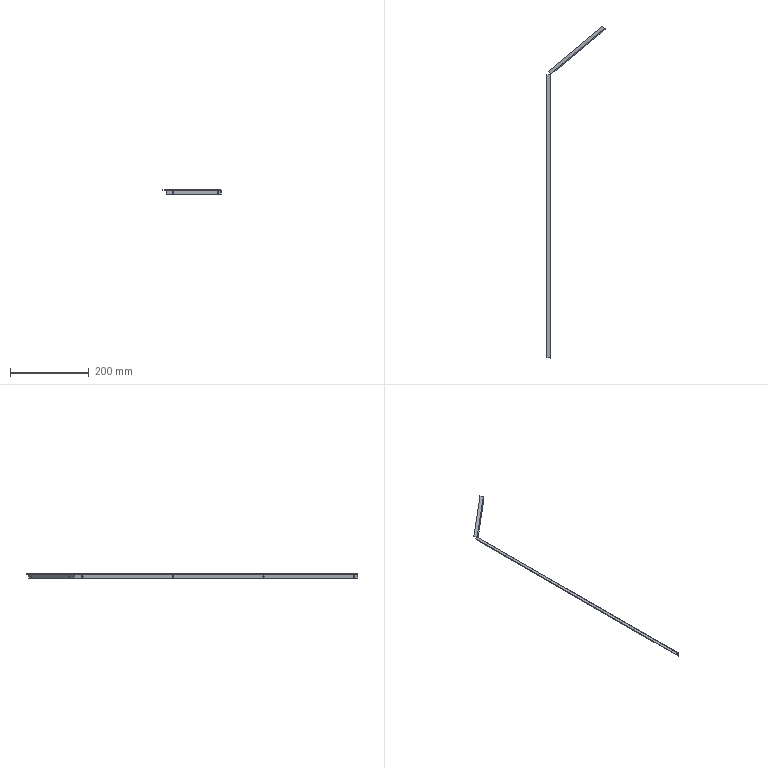Component | SolidWorks | SYM0671-81-200-1_SYM0671-81-202-1 | 1 solid | 44 faces | volume 8722 mm3 | plane 26 | cylinder 18 | commonest cylinder face diameters 3.5 x12 3 x3 2 x3 | material AISI 304